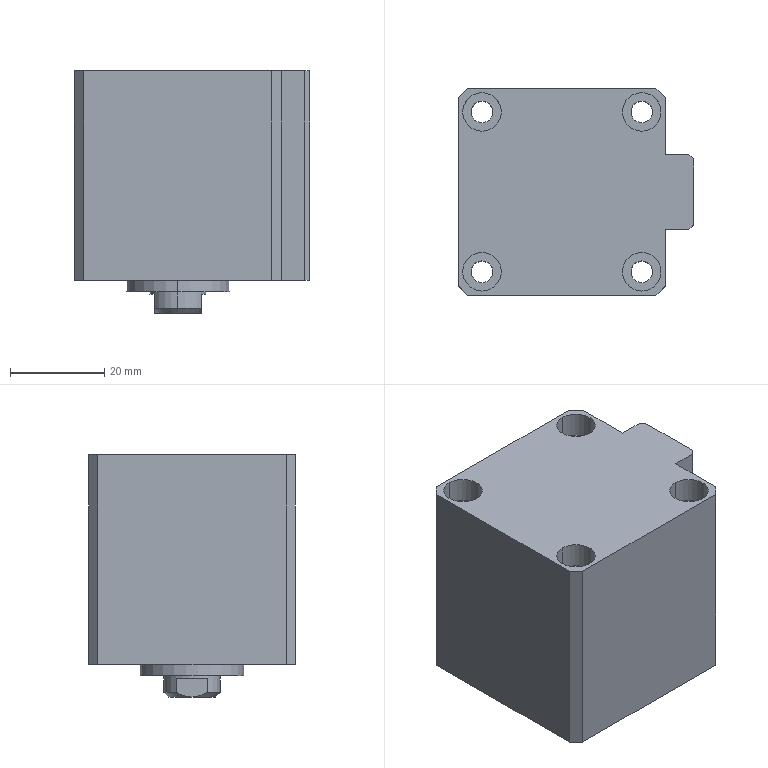Component | SolidWorks | DirectPressureVerticalSeal-1_SDA32X20-1 | 1 solid | 81 faces | volume 85321 mm3 | cylinder 34 | plane 32 | cone 15 | commonest cylinder face diameters 8.2 x16 4.6 x8 7.9 x4 22 x2 12 x2 6.8 x2